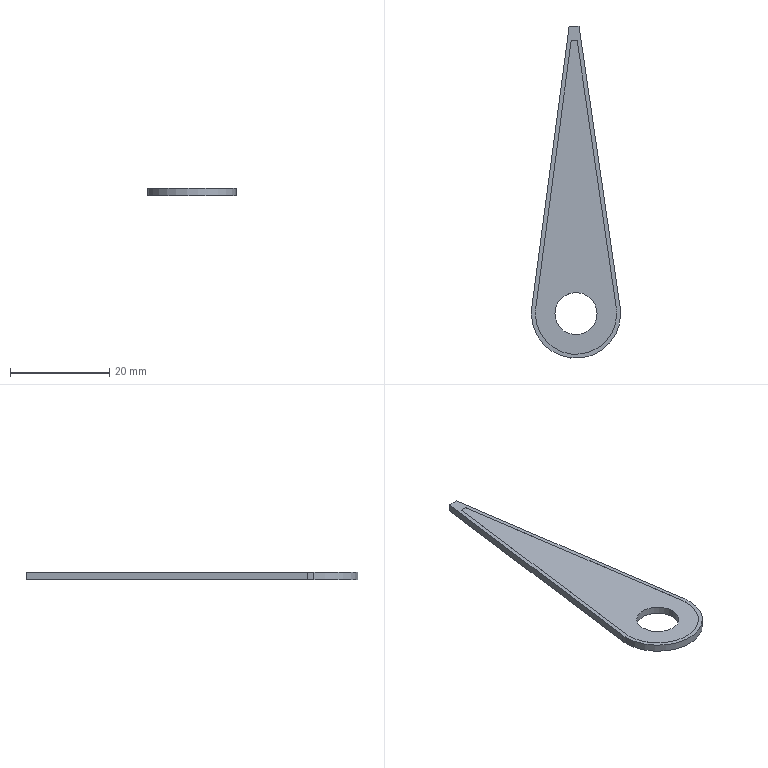Component | SolidWorks | JF21-80.2-14-1-SOLID1-1 | 1 solid | 17 faces | box 18 x 67.01 x 1.5 mm | volume 982 mm3 | plane 9 | cylinder 8 | commonest cylinder face diameters 16.4 x3 18 x3 8.5 x2
STEP:
#1=COLOUR_RGB('',0.7922,0.8196,0.9333);
#2=FILL_AREA_STYLE_COLOUR('',#1);
#3=FILL_AREA_STYLE('',(#2));
#4=SURFACE_STYLE_FILL_AREA(#3);
#5=SURFACE_SIDE_STYLE('',(#4));
#6=SURFACE_STYLE_USAGE(.BOTH.,#5);
#7=PRESENTATION_STYLE_ASSIGNMENT((#6));
#8=CARTESIAN_POINT('',(-0.32,0.03262,-13.268));
#9=VERTEX_POINT('',#8);
#10=CARTESIAN_POINT('',(-0.3228,-0.01198,-13.268));
#11=VERTEX_POINT('',#10);
#12=CARTESIAN_POINT('',(-0.,-0.009843,-13.268));
#13=DIRECTION('',(0.,0.,1.));
#14=DIRECTION('',(1.,0.006635,0.));
#15=AXIS2_PLACEMENT_3D('',#12,#13,#14);
#16=CIRCLE('',#15,0.3228);
#17=EDGE_CURVE('',#9,#11,#16,.T.);
#18=ORIENTED_EDGE('',*,*,#17,.T.);
#19=CARTESIAN_POINT('',(-0.3228,-0.01198,-13.268));
#20=VERTEX_POINT('',#19);
#21=CARTESIAN_POINT('',(-0.3228,-0.01198,-13.268));
#22=DIRECTION('',(0.,0.,1.));
#23=VECTOR('',#22,39.37);
#24=LINE('',#21,#23);
#25=EDGE_CURVE('',#11,#20,#24,.T.);
#26=ORIENTED_EDGE('',*,*,#25,.T.);
#27=CARTESIAN_POINT('',(-0.32,0.03262,-13.268));
#28=VERTEX_POINT('',#27);
#29=CARTESIAN_POINT('',(-0.,-0.009843,-13.268));
#30=DIRECTION('',(0.,0.,1.));
#31=DIRECTION('',(1.,0.006635,0.));
#32=AXIS2_PLACEMENT_3D('',#29,#30,#31);
#33=CIRCLE('',#32,0.3228);
#34=EDGE_CURVE('',#28,#20,#33,.T.);
#35=ORIENTED_EDGE('',*,*,#34,.F.);
#36=CARTESIAN_POINT('',(-0.32,0.03262,-13.268));
#37=DIRECTION('',(0.,0.,1.));
#38=VECTOR('',#37,39.37);
#39=LINE('',#36,#38);
#40=EDGE_CURVE('',#9,#28,#39,.T.);
#41=ORIENTED_EDGE('',*,*,#40,.F.);
#42=EDGE_LOOP('',(#18,#26,#35,#41));
#43=FACE_OUTER_BOUND('',#42,.T.);
#44=CARTESIAN_POINT('',(-0.,-0.009843,-13.268));
#45=DIRECTION('',(0.,0.,1.));
#46=DIRECTION('',(-1.,-0.006635,0.));
#47=AXIS2_PLACEMENT_3D('',#44,#45,#46);
#48=CYLINDRICAL_SURFACE('',#47,0.3228);
#49=ADVANCED_FACE('',(#43),#48,.T.);
#50=ORIENTED_EDGE('',*,*,#25,.F.);
#51=CARTESIAN_POINT('',(0.3228,-0.0077,-13.268));
#52=VERTEX_POINT('',#51);
#53=CARTESIAN_POINT('',(-0.,-0.009843,-13.268));
#54=DIRECTION('',(0.,0.,1.));
#55=DIRECTION('',(1.,0.006635,0.));
#56=AXIS2_PLACEMENT_3D('',#53,#54,#55);
#57=CIRCLE('',#56,0.3228);
#58=EDGE_CURVE('',#11,#52,#57,.T.);
#59=ORIENTED_EDGE('',*,*,#58,.T.);
#60=CARTESIAN_POINT('',(0.3228,-0.0077,-13.268));
#61=VERTEX_POINT('',#60);
#62=CARTESIAN_POINT('',(0.3228,-0.0077,-13.268));
#63=DIRECTION('',(0.,0.,1.));
#64=VECTOR('',#63,39.37);
#65=LINE('',#62,#64);
#66=EDGE_CURVE('',#52,#61,#65,.T.);
#67=ORIENTED_EDGE('',*,*,#66,.T.);
#68=CARTESIAN_POINT('',(-0.,-0.009843,-13.268));
#69=DIRECTION('',(0.,0.,1.));
#70=DIRECTION('',(1.,0.006635,0.));
#71=AXIS2_PLACEMENT_3D('',#68,#69,#70);
#72=CIRCLE('',#71,0.3228);
#73=EDGE_CURVE('',#20,#61,#72,.T.);
#74=ORIENTED_EDGE('',*,*,#73,.F.);
#75=EDGE_LOOP('',(#50,#59,#67,#74));
#76=FACE_OUTER_BOUND('',#75,.T.);
#77=CARTESIAN_POINT('',(-0.,-0.009843,-13.268));
#78=DIRECTION('',(0.,0.,1.));
#79=DIRECTION('',(-1.,-0.006635,0.));
#80=AXIS2_PLACEMENT_3D('',#77,#78,#79);
#81=CYLINDRICAL_SURFACE('',#80,0.3228);
#82=ADVANCED_FACE('',(#76),#81,.T.);
#83=CARTESIAN_POINT('',(-0.1673,-0.01095,-13.327));
#84=VERTEX_POINT('',#83);
#85=CARTESIAN_POINT('',(0.1673,-0.008732,-13.327));
#86=VERTEX_POINT('',#85);
#87=CARTESIAN_POINT('',(-0.,-0.009843,-13.327));
#88=DIRECTION('',(0.,0.,1.));
#89=DIRECTION('',(1.,0.006635,0.));
#90=AXIS2_PLACEMENT_3D('',#87,#88,#89);
#91=CIRCLE('',#90,0.1673);
#92=EDGE_CURVE('',#84,#86,#91,.T.);
#93=ORIENTED_EDGE('',*,*,#92,.F.);
#94=CARTESIAN_POINT('',(-0.1673,-0.01095,-13.268));
#95=VERTEX_POINT('',#94);
#96=CARTESIAN_POINT('',(-0.1673,-0.01095,-13.327));
#97=DIRECTION('',(0.,0.,1.));
#98=VECTOR('',#97,39.37);
#99=LINE('',#96,#98);
#100=EDGE_CURVE('',#84,#95,#99,.T.);
#101=ORIENTED_EDGE('',*,*,#100,.T.);
#102=CARTESIAN_POINT('',(0.1673,-0.008732,-13.268));
#103=VERTEX_POINT('',#102);
#104=CARTESIAN_POINT('',(-0.,-0.009843,-13.268));
#105=DIRECTION('',(0.,0.,1.));
#106=DIRECTION('',(1.,0.006635,0.));
#107=AXIS2_PLACEMENT_3D('',#104,#105,#106);
#108=CIRCLE('',#107,0.1673);
#109=EDGE_CURVE('',#95,#103,#108,.T.);
#110=ORIENTED_EDGE('',*,*,#109,.T.);
#111=CARTESIAN_POINT('',(0.1673,-0.008732,-13.327));
#112=DIRECTION('',(0.,0.,1.));
#113=VECTOR('',#112,39.37);
#114=LINE('',#111,#113);
#115=EDGE_CURVE('',#86,#103,#114,.T.);
#116=ORIENTED_EDGE('',*,*,#115,.F.);
#117=EDGE_LOOP('',(#93,#101,#110,#116));
#118=FACE_OUTER_BOUND('',#117,.T.);
#119=CARTESIAN_POINT('',(-0.,-0.009843,-13.327));
#120=DIRECTION('',(0.,0.,1.));
#121=DIRECTION('',(-1.,-0.006635,0.));
#122=AXIS2_PLACEMENT_3D('',#119,#120,#121);
#123=CYLINDRICAL_SURFACE('',#122,0.1673);
#124=ADVANCED_FACE('',(#118),#123,.F.);
#125=CARTESIAN_POINT('',(0.3543,-0.007491,-13.268));
#126=VERTEX_POINT('',#125);
#127=CARTESIAN_POINT('',(0.3506,0.04142,-13.268));
#128=VERTEX_POINT('',#127);
#129=CARTESIAN_POINT('',(-0.,-0.009843,-13.268));
#130=DIRECTION('',(0.,0.,1.));
#131=DIRECTION('',(1.,0.006635,0.));
#132=AXIS2_PLACEMENT_3D('',#129,#130,#131);
#133=CIRCLE('',#132,0.3543);
#134=EDGE_CURVE('',#126,#128,#133,.T.);
#135=ORIENTED_EDGE('',*,*,#134,.F.);
#136=CARTESIAN_POINT('',(0.3543,-0.007491,-13.327));
#137=VERTEX_POINT('',#136);
#138=CARTESIAN_POINT('',(0.3543,-0.007491,-13.268));
#139=DIRECTION('',(0.,0.,-1.));
#140=VECTOR('',#139,39.37);
#141=LINE('',#138,#140);
#142=EDGE_CURVE('',#126,#137,#141,.T.);
#143=ORIENTED_EDGE('',*,*,#142,.T.);
#144=CARTESIAN_POINT('',(0.3506,0.04142,-13.327));
#145=VERTEX_POINT('',#144);
#146=CARTESIAN_POINT('',(-0.,-0.009843,-13.327));
#147=DIRECTION('',(0.,0.,1.));
#148=DIRECTION('',(1.,0.006635,0.));
#149=AXIS2_PLACEMENT_3D('',#146,#147,#148);
#150=CIRCLE('',#149,0.3543);
#151=EDGE_CURVE('',#137,#145,#150,.T.);
#152=ORIENTED_EDGE('',*,*,#151,.T.);
#153=CARTESIAN_POINT('',(0.3506,0.04142,-13.268));
#154=DIRECTION('',(0.,0.,-1.));
#155=VECTOR('',#154,39.37);
#156=LINE('',#153,#155);
#157=EDGE_CURVE('',#128,#145,#156,.T.);
#158=ORIENTED_EDGE('',*,*,#157,.F.);
#159=EDGE_LOOP('',(#135,#143,#152,#158));
#160=FACE_OUTER_BOUND('',#159,.T.);
#161=CARTESIAN_POINT('',(-0.,-0.009843,-13.268));
#162=DIRECTION('',(0.,0.,-1.));
#163=DIRECTION('',(1.,0.006635,0.));
#164=AXIS2_PLACEMENT_3D('',#161,#162,#163);
#165=CYLINDRICAL_SURFACE('',#164,0.3543);
#166=ADVANCED_FACE('',(#160),#165,.T.);
#167=ORIENTED_EDGE('',*,*,#142,.F.);
#168=CARTESIAN_POINT('',(-0.3543,-0.01219,-13.268));
#169=VERTEX_POINT('',#168);
#170=CARTESIAN_POINT('',(-0.,-0.009843,-13.268));
#171=DIRECTION('',(0.,0.,1.));
#172=DIRECTION('',(1.,0.006635,0.));
#173=AXIS2_PLACEMENT_3D('',#170,#171,#172);
#174=CIRCLE('',#173,0.3543);
#175=EDGE_CURVE('',#169,#126,#174,.T.);
#176=ORIENTED_EDGE('',*,*,#175,.F.);
#177=CARTESIAN_POINT('',(-0.3543,-0.01219,-13.327));
#178=VERTEX_POINT('',#177);
#179=CARTESIAN_POINT('',(-0.3543,-0.01219,-13.268));
#180=DIRECTION('',(0.,0.,-1.));
#181=VECTOR('',#180,39.37);
#182=LINE('',#179,#181);
#183=EDGE_CURVE('',#169,#178,#182,.T.);
#184=ORIENTED_EDGE('',*,*,#183,.T.);
#185=CARTESIAN_POINT('',(-0.,-0.009843,-13.327));
#186=DIRECTION('',(0.,0.,1.));
#187=DIRECTION('',(1.,0.006635,0.));
#188=AXIS2_PLACEMENT_3D('',#185,#186,#187);
#189=CIRCLE('',#188,0.3543);
#190=EDGE_CURVE('',#178,#137,#189,.T.);
#191=ORIENTED_EDGE('',*,*,#190,.T.);
#192=EDGE_LOOP('',(#167,#176,#184,#191));
#193=FACE_OUTER_BOUND('',#192,.T.);
#194=CARTESIAN_POINT('',(-0.,-0.009843,-13.268));
#195=DIRECTION('',(0.,0.,-1.));
#196=DIRECTION('',(1.,0.006635,0.));
#197=AXIS2_PLACEMENT_3D('',#194,#195,#196);
#198=CYLINDRICAL_SURFACE('',#197,0.3543);
#199=ADVANCED_FACE('',(#193),#198,.T.);
#200=CARTESIAN_POINT('',(-0.05452,2.273,-13.268));
#201=VERTEX_POINT('',#200);
#202=CARTESIAN_POINT('',(-0.3513,0.03676,-13.268));
#203=VERTEX_POINT('',#202);
#204=CARTESIAN_POINT('',(-0.05452,2.273,-13.268));
#205=DIRECTION('',(-0.1315,-0.9913,0.));
#206=VECTOR('',#205,39.37);
#207=LINE('',#204,#206);
#208=EDGE_CURVE('',#201,#203,#207,.T.);
#209=ORIENTED_EDGE('',*,*,#208,.F.);
#210=CARTESIAN_POINT('',(-0.05452,2.273,-13.327));
#211=VERTEX_POINT('',#210);
#212=CARTESIAN_POINT('',(-0.05452,2.273,-13.268));
#213=DIRECTION('',(0.,0.,-1.));
#214=VECTOR('',#213,39.37);
#215=LINE('',#212,#214);
#216=EDGE_CURVE('',#201,#211,#215,.T.);
#217=ORIENTED_EDGE('',*,*,#216,.T.);
#218=CARTESIAN_POINT('',(-0.3513,0.03676,-13.327));
#219=VERTEX_POINT('',#218);
#220=CARTESIAN_POINT('',(-0.05452,2.273,-13.327));
#221=DIRECTION('',(-0.1315,-0.9913,0.));
#222=VECTOR('',#221,39.37);
#223=LINE('',#220,#222);
#224=EDGE_CURVE('',#211,#219,#223,.T.);
#225=ORIENTED_EDGE('',*,*,#224,.T.);
#226=CARTESIAN_POINT('',(-0.3513,0.03676,-13.268));
#227=DIRECTION('',(0.,0.,-1.));
#228=VECTOR('',#227,39.37);
#229=LINE('',#226,#228);
#230=EDGE_CURVE('',#203,#219,#229,.T.);
#231=ORIENTED_EDGE('',*,*,#230,.F.);
#232=EDGE_LOOP('',(#209,#217,#225,#231));
#233=FACE_OUTER_BOUND('',#232,.T.);
#234=CARTESIAN_POINT('',(-0.05452,2.273,-13.268));
#235=DIRECTION('',(0.9913,-0.1315,0.));
#236=DIRECTION('',(-0.1315,-0.9913,0.));
#237=AXIS2_PLACEMENT_3D('',#234,#235,#236);
#238=PLANE('',#237);
#239=ADVANCED_FACE('',(#233),#238,.F.);
#240=ORIENTED_EDGE('',*,*,#183,.F.);
#241=CARTESIAN_POINT('',(-0.,-0.009843,-13.268));
#242=DIRECTION('',(0.,0.,1.));
#243=DIRECTION('',(1.,0.006635,0.));
#244=AXIS2_PLACEMENT_3D('',#241,#242,#243);
#245=CIRCLE('',#244,0.3543);
#246=EDGE_CURVE('',#203,#169,#245,.T.);
#247=ORIENTED_EDGE('',*,*,#246,.F.);
#248=ORIENTED_EDGE('',*,*,#230,.T.);
#249=CARTESIAN_POINT('',(-0.,-0.009843,-13.327));
#250=DIRECTION('',(0.,0.,1.));
#251=DIRECTION('',(1.,0.006635,0.));
#252=AXIS2_PLACEMENT_3D('',#249,#250,#251);
#253=CIRCLE('',#252,0.3543);
#254=EDGE_CURVE('',#219,#178,#253,.T.);
#255=ORIENTED_EDGE('',*,*,#254,.T.);
#256=EDGE_LOOP('',(#240,#247,#248,#255));
#257=FACE_OUTER_BOUND('',#256,.T.);
#258=CARTESIAN_POINT('',(-0.,-0.009843,-13.268));
#259=DIRECTION('',(0.,0.,-1.));
#260=DIRECTION('',(1.,0.006635,0.));
#261=AXIS2_PLACEMENT_3D('',#258,#259,#260);
#262=CYLINDRICAL_SURFACE('',#261,0.3543);
#263=ADVANCED_FACE('',(#257),#262,.T.);
#264=CARTESIAN_POINT('',(0.02422,2.274,-13.268));
#265=VERTEX_POINT('',#264);
#266=CARTESIAN_POINT('',(0.02422,2.274,-13.268));
#267=DIRECTION('',(-0.1447,0.9895,0.));
#268=VECTOR('',#267,39.37);
#269=LINE('',#266,#268);
#270=EDGE_CURVE('',#128,#265,#269,.T.);
#271=ORIENTED_EDGE('',*,*,#270,.F.);
#272=ORIENTED_EDGE('',*,*,#157,.T.);
#273=CARTESIAN_POINT('',(0.02422,2.274,-13.327));
#274=VERTEX_POINT('',#273);
#275=CARTESIAN_POINT('',(0.02422,2.274,-13.327));
#276=DIRECTION('',(-0.1447,0.9895,0.));
#277=VECTOR('',#276,39.37);
#278=LINE('',#275,#277);
#279=EDGE_CURVE('',#145,#274,#278,.T.);
#280=ORIENTED_EDGE('',*,*,#279,.T.);
#281=CARTESIAN_POINT('',(0.02422,2.274,-13.268));
#282=DIRECTION('',(0.,0.,-1.));
#283=VECTOR('',#282,39.37);
#284=LINE('',#281,#283);
#285=EDGE_CURVE('',#265,#274,#284,.T.);
#286=ORIENTED_EDGE('',*,*,#285,.F.);
#287=EDGE_LOOP('',(#271,#272,#280,#286));
#288=FACE_OUTER_BOUND('',#287,.T.);
#289=CARTESIAN_POINT('',(0.02422,2.274,-13.268));
#290=DIRECTION('',(-0.9895,-0.1447,0.));
#291=DIRECTION('',(-0.1447,0.9895,0.));
#292=AXIS2_PLACEMENT_3D('',#289,#290,#291);
#293=PLANE('',#292);
#294=ADVANCED_FACE('',(#288),#293,.F.);
#295=CARTESIAN_POINT('',(-0.05452,2.273,-13.268));
#296=DIRECTION('',(-1.,-0.006635,0.));
#297=VECTOR('',#296,39.37);
#298=LINE('',#295,#297);
#299=EDGE_CURVE('',#265,#201,#298,.T.);
#300=ORIENTED_EDGE('',*,*,#299,.F.);
#301=ORIENTED_EDGE('',*,*,#285,.T.);
#302=CARTESIAN_POINT('',(-0.05452,2.273,-13.327));
#303=DIRECTION('',(-1.,-0.006635,0.));
#304=VECTOR('',#303,39.37);
#305=LINE('',#302,#304);
#306=EDGE_CURVE('',#274,#211,#305,.T.);
#307=ORIENTED_EDGE('',*,*,#306,.T.);
#308=ORIENTED_EDGE('',*,*,#216,.F.);
#309=EDGE_LOOP('',(#300,#301,#307,#308));
#310=FACE_OUTER_BOUND('',#309,.T.);
#311=CARTESIAN_POINT('',(-0.05452,2.273,-13.268));
#312=DIRECTION('',(0.006635,-1.,0.));
#313=DIRECTION('',(0.,0.,1.));
#314=AXIS2_PLACEMENT_3D('',#311,#312,#313);
#315=PLANE('',#314);
#316=ADVANCED_FACE('',(#310),#315,.F.);
#317=CARTESIAN_POINT('',(-0.,-0.009843,-13.268));
#318=DIRECTION('',(0.,0.,1.));
#319=DIRECTION('',(1.,0.006635,0.));
#320=AXIS2_PLACEMENT_3D('',#317,#318,#319);
#321=CIRCLE('',#320,0.1673);
#322=EDGE_CURVE('',#103,#95,#321,.T.);
#323=ORIENTED_EDGE('',*,*,#322,.F.);
#324=ORIENTED_EDGE('',*,*,#109,.F.);
#325=EDGE_LOOP('',(#323,#324));
#326=FACE_BOUND('',#325,.T.);
#327=ORIENTED_EDGE('',*,*,#34,.T.);
#328=ORIENTED_EDGE('',*,*,#73,.T.);
#329=CARTESIAN_POINT('',(0.3194,0.03686,-13.268));
#330=VERTEX_POINT('',#329);
#331=CARTESIAN_POINT('',(-0.,-0.009843,-13.268));
#332=DIRECTION('',(0.,0.,1.));
#333=DIRECTION('',(1.,0.006635,0.));
#334=AXIS2_PLACEMENT_3D('',#331,#332,#333);
#335=CIRCLE('',#334,0.3228);
#336=EDGE_CURVE('',#61,#330,#335,.T.);
#337=ORIENTED_EDGE('',*,*,#336,.T.);
#338=CARTESIAN_POINT('',(0.009669,2.156,-13.268));
#339=VERTEX_POINT('',#338);
#340=CARTESIAN_POINT('',(0.3194,0.03686,-13.268));
#341=DIRECTION('',(-0.1447,0.9895,0.));
#342=VECTOR('',#341,39.37);
#343=LINE('',#340,#342);
#344=EDGE_CURVE('',#330,#339,#343,.T.);
#345=ORIENTED_EDGE('',*,*,#344,.T.);
#346=CARTESIAN_POINT('',(-0.03841,2.155,-13.268));
#347=VERTEX_POINT('',#346);
#348=CARTESIAN_POINT('',(-0.03841,2.155,-13.268));
#349=DIRECTION('',(-1.,-0.006635,0.));
#350=VECTOR('',#349,39.37);
#351=LINE('',#348,#350);
#352=EDGE_CURVE('',#339,#347,#351,.T.);
#353=ORIENTED_EDGE('',*,*,#352,.T.);
#354=CARTESIAN_POINT('',(-0.03841,2.155,-13.268));
#355=DIRECTION('',(-0.1315,-0.9913,0.));
#356=VECTOR('',#355,39.37);
#357=LINE('',#354,#356);
#358=EDGE_CURVE('',#347,#28,#357,.T.);
#359=ORIENTED_EDGE('',*,*,#358,.T.);
#360=EDGE_LOOP('',(#327,#328,#337,#345,#353,#359));
#361=FACE_OUTER_BOUND('',#360,.T.);
#362=CARTESIAN_POINT('',(-0.,-0.009843,-13.268));
#363=DIRECTION('',(0.,0.,1.));
#364=DIRECTION('',(-1.,-0.006635,0.));
#365=AXIS2_PLACEMENT_3D('',#362,#363,#364);
#366=PLANE('',#365);
#367=ADVANCED_FACE('',(#326,#361),#366,.T.);
#368=CARTESIAN_POINT('',(-0.,-0.009843,-13.327));
#369=DIRECTION('',(0.,0.,1.));
#370=DIRECTION('',(1.,0.006635,0.));
#371=AXIS2_PLACEMENT_3D('',#368,#369,#370);
#372=CIRCLE('',#371,0.1673);
#373=EDGE_CURVE('',#86,#84,#372,.T.);
#374=ORIENTED_EDGE('',*,*,#373,.T.);
#375=ORIENTED_EDGE('',*,*,#92,.T.);
#376=EDGE_LOOP('',(#374,#375));
#377=FACE_BOUND('',#376,.T.);
#378=ORIENTED_EDGE('',*,*,#224,.F.);
#379=ORIENTED_EDGE('',*,*,#306,.F.);
#380=ORIENTED_EDGE('',*,*,#279,.F.);
#381=ORIENTED_EDGE('',*,*,#151,.F.);
#382=ORIENTED_EDGE('',*,*,#190,.F.);
#383=ORIENTED_EDGE('',*,*,#254,.F.);
#384=EDGE_LOOP('',(#378,#379,#380,#381,#382,#383));
#385=FACE_OUTER_BOUND('',#384,.T.);
#386=CARTESIAN_POINT('',(-0.,-0.009843,-13.327));
#387=DIRECTION('',(0.,0.,1.));
#388=DIRECTION('',(-1.,-0.006635,0.));
#389=AXIS2_PLACEMENT_3D('',#386,#387,#388);
#390=PLANE('',#389);
#391=ADVANCED_FACE('',(#377,#385),#390,.F.);
#392=ORIENTED_EDGE('',*,*,#100,.F.);
#393=ORIENTED_EDGE('',*,*,#373,.F.);
#394=ORIENTED_EDGE('',*,*,#115,.T.);
#395=ORIENTED_EDGE('',*,*,#322,.T.);
#396=EDGE_LOOP('',(#392,#393,#394,#395));
#397=FACE_OUTER_BOUND('',#396,.T.);
#398=CARTESIAN_POINT('',(-0.,-0.009843,-13.327));
#399=DIRECTION('',(0.,0.,1.));
#400=DIRECTION('',(-1.,-0.006635,0.));
#401=AXIS2_PLACEMENT_3D('',#398,#399,#400);
#402=CYLINDRICAL_SURFACE('',#401,0.1673);
#403=ADVANCED_FACE('',(#397),#402,.F.);
#404=ORIENTED_EDGE('',*,*,#17,.F.);
#405=CARTESIAN_POINT('',(-0.03841,2.155,-13.268));
#406=VERTEX_POINT('',#405);
#407=CARTESIAN_POINT('',(-0.03841,2.155,-13.268));
#408=DIRECTION('',(-0.1315,-0.9913,0.));
#409=VECTOR('',#408,39.37);
#410=LINE('',#407,#409);
#411=EDGE_CURVE('',#406,#9,#410,.T.);
#412=ORIENTED_EDGE('',*,*,#411,.F.);
#413=CARTESIAN_POINT('',(0.009669,2.156,-13.268));
#414=VERTEX_POINT('',#413);
#415=CARTESIAN_POINT('',(-0.03841,2.155,-13.268));
#416=DIRECTION('',(-1.,-0.006635,0.));
#417=VECTOR('',#416,39.37);
#418=LINE('',#415,#417);
#419=EDGE_CURVE('',#414,#406,#418,.T.);
#420=ORIENTED_EDGE('',*,*,#419,.F.);
#421=CARTESIAN_POINT('',(0.3194,0.03686,-13.268));
#422=VERTEX_POINT('',#421);
#423=CARTESIAN_POINT('',(0.3194,0.03686,-13.268));
#424=DIRECTION('',(-0.1447,0.9895,0.));
#425=VECTOR('',#424,39.37);
#426=LINE('',#423,#425);
#427=EDGE_CURVE('',#422,#414,#426,.T.);
#428=ORIENTED_EDGE('',*,*,#427,.F.);
#429=CARTESIAN_POINT('',(-0.,-0.009843,-13.268));
#430=DIRECTION('',(0.,0.,1.));
#431=DIRECTION('',(1.,0.006635,0.));
#432=AXIS2_PLACEMENT_3D('',#429,#430,#431);
#433=CIRCLE('',#432,0.3228);
#434=EDGE_CURVE('',#52,#422,#433,.T.);
#435=ORIENTED_EDGE('',*,*,#434,.F.);
#436=ORIENTED_EDGE('',*,*,#58,.F.);
#437=EDGE_LOOP('',(#404,#412,#420,#428,#435,#436));
#438=FACE_BOUND('',#437,.T.);
#439=ORIENTED_EDGE('',*,*,#208,.T.);
#440=ORIENTED_EDGE('',*,*,#246,.T.);
#441=ORIENTED_EDGE('',*,*,#175,.T.);
#442=ORIENTED_EDGE('',*,*,#134,.T.);
#443=ORIENTED_EDGE('',*,*,#270,.T.);
#444=ORIENTED_EDGE('',*,*,#299,.T.);
#445=EDGE_LOOP('',(#439,#440,#441,#442,#443,#444));
#446=FACE_OUTER_BOUND('',#445,.T.);
#447=CARTESIAN_POINT('',(-0.0064,0.9547,-13.268));
#448=DIRECTION('',(0.,0.,1.));
#449=DIRECTION('',(-1.,-0.006635,0.));
#450=AXIS2_PLACEMENT_3D('',#447,#448,#449);
#451=PLANE('',#450);
#452=ADVANCED_FACE('',(#438,#446),#451,.T.);
#453=ORIENTED_EDGE('',*,*,#344,.F.);
#454=CARTESIAN_POINT('',(0.3194,0.03686,-13.268));
#455=DIRECTION('',(0.,0.,1.));
#456=VECTOR('',#455,39.37);
#457=LINE('',#454,#456);
#458=EDGE_CURVE('',#422,#330,#457,.T.);
#459=ORIENTED_EDGE('',*,*,#458,.F.);
#460=ORIENTED_EDGE('',*,*,#427,.T.);
#461=CARTESIAN_POINT('',(0.009669,2.156,-13.268));
#462=DIRECTION('',(0.,0.,1.));
#463=VECTOR('',#462,39.37);
#464=LINE('',#461,#463);
#465=EDGE_CURVE('',#414,#339,#464,.T.);
#466=ORIENTED_EDGE('',*,*,#465,.T.);
#467=EDGE_LOOP('',(#453,#459,#460,#466));
#468=FACE_OUTER_BOUND('',#467,.T.);
#469=CARTESIAN_POINT('',(0.3194,0.03686,-13.268));
#470=DIRECTION('',(0.9895,0.1447,0.));
#471=DIRECTION('',(0.1447,-0.9895,0.));
#472=AXIS2_PLACEMENT_3D('',#469,#470,#471);
#473=PLANE('',#472);
#474=ADVANCED_FACE('',(#468),#473,.T.);
#475=ORIENTED_EDGE('',*,*,#66,.F.);
#476=ORIENTED_EDGE('',*,*,#434,.T.);
#477=ORIENTED_EDGE('',*,*,#458,.T.);
#478=ORIENTED_EDGE('',*,*,#336,.F.);
#479=EDGE_LOOP('',(#475,#476,#477,#478));
#480=FACE_OUTER_BOUND('',#479,.T.);
#481=CARTESIAN_POINT('',(-0.,-0.009843,-13.268));
#482=DIRECTION('',(0.,0.,1.));
#483=DIRECTION('',(-1.,-0.006635,0.));
#484=AXIS2_PLACEMENT_3D('',#481,#482,#483);
#485=CYLINDRICAL_SURFACE('',#484,0.3228);
#486=ADVANCED_FACE('',(#480),#485,.T.);
#487=ORIENTED_EDGE('',*,*,#358,.F.);
#488=CARTESIAN_POINT('',(-0.03841,2.155,-13.268));
#489=DIRECTION('',(0.,0.,1.));
#490=VECTOR('',#489,39.37);
#491=LINE('',#488,#490);
#492=EDGE_CURVE('',#406,#347,#491,.T.);
#493=ORIENTED_EDGE('',*,*,#492,.F.);
#494=ORIENTED_EDGE('',*,*,#411,.T.);
#495=ORIENTED_EDGE('',*,*,#40,.T.);
#496=EDGE_LOOP('',(#487,#493,#494,#495));
#497=FACE_OUTER_BOUND('',#496,.T.);
#498=CARTESIAN_POINT('',(-0.03841,2.155,-13.268));
#499=DIRECTION('',(-0.9913,0.1315,0.));
#500=DIRECTION('',(0.1315,0.9913,0.));
#501=AXIS2_PLACEMENT_3D('',#498,#499,#500);
#502=PLANE('',#501);
#503=ADVANCED_FACE('',(#497),#502,.T.);
#504=ORIENTED_EDGE('',*,*,#352,.F.);
#505=ORIENTED_EDGE('',*,*,#465,.F.);
#506=ORIENTED_EDGE('',*,*,#419,.T.);
#507=ORIENTED_EDGE('',*,*,#492,.T.);
#508=EDGE_LOOP('',(#504,#505,#506,#507));
#509=FACE_OUTER_BOUND('',#508,.T.);
#510=CARTESIAN_POINT('',(-0.03841,2.155,-13.268));
#511=DIRECTION('',(-0.006635,1.,0.));
#512=DIRECTION('',(0.,0.,-1.));
#513=AXIS2_PLACEMENT_3D('',#510,#511,#512);
#514=PLANE('',#513);
#515=ADVANCED_FACE('',(#509),#514,.T.);
#516=CLOSED_SHELL('',(#49,#82,#124,#166,#199,#239,#263,#294,#316,#367,#391,#403,#452,#474,#486,#503,#515));
#517=MANIFOLD_SOLID_BREP('',#516);
#518=STYLED_ITEM('',(#7),#517);
#519=PRESENTATION_LAYER_ASSIGNMENT('','',(#518));
#520=(LENGTH_UNIT()NAMED_UNIT(*)SI_UNIT($,.METRE.));
#521=LENGTH_MEASURE_WITH_UNIT(LENGTH_MEASURE(0.0254),#520);
#522=DIMENSIONAL_EXPONENTS(1.,0.,0.,0.,0.,0.,0.);
#523=(CONVERSION_BASED_UNIT('',#521)LENGTH_UNIT()NAMED_UNIT(#522));
#524=UNCERTAINTY_MEASURE_WITH_UNIT(LENGTH_MEASURE(0.00001),#523,'','');
#525=(NAMED_UNIT(*)PLANE_ANGLE_UNIT()SI_UNIT($,.RADIAN.));
#526=(NAMED_UNIT(*)SI_UNIT($,.STERADIAN.)SOLID_ANGLE_UNIT());
#527=(GEOMETRIC_REPRESENTATION_CONTEXT(3)GLOBAL_UNCERTAINTY_ASSIGNED_CONTEXT((#524))GLOBAL_UNIT_ASSIGNED_CONTEXT((#523,#525,#526))REPRESENTATION_CONTEXT('',''));
#528=MECHANICAL_DESIGN_GEOMETRIC_PRESENTATION_REPRESENTATION('',(#518),#527);
#529=CARTESIAN_POINT('',(0.,0.,0.));
#530=DIRECTION('',(0.,0.,1.));
#531=DIRECTION('',(1.,0.,0.));
#532=AXIS2_PLACEMENT_3D('',#529,#530,#531);
#533=(LENGTH_UNIT()NAMED_UNIT(*)SI_UNIT($,.METRE.));
#534=LENGTH_MEASURE_WITH_UNIT(LENGTH_MEASURE(0.0254),#533);
#535=DIMENSIONAL_EXPONENTS(1.,0.,0.,0.,0.,0.,0.);
#536=(CONVERSION_BASED_UNIT('',#534)LENGTH_UNIT()NAMED_UNIT(#535));
#537=UNCERTAINTY_MEASURE_WITH_UNIT(LENGTH_MEASURE(0.00001),#536,'','');
#538=(NAMED_UNIT(*)PLANE_ANGLE_UNIT()SI_UNIT($,.RADIAN.));
#539=(NAMED_UNIT(*)SI_UNIT($,.STERADIAN.)SOLID_ANGLE_UNIT());
#540=(GEOMETRIC_REPRESENTATION_CONTEXT(3)GLOBAL_UNCERTAINTY_ASSIGNED_CONTEXT((#537))GLOBAL_UNIT_ASSIGNED_CONTEXT((#536,#538,#539))REPRESENTATION_CONTEXT('',''));
#541=ADVANCED_BREP_SHAPE_REPRESENTATION('',(#517,#532),#540);